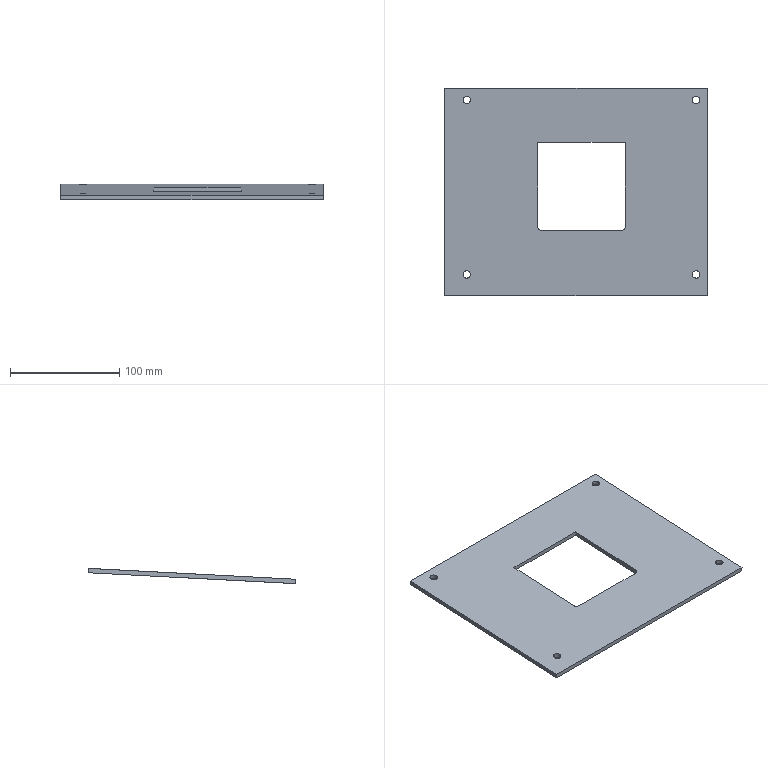Component | SolidWorks | YC1-250HangingBoxOverall-1_YC1-250SupportBracketT()-1_YC1-160OperationStationBaffleT-1 | 1 solid | 20 faces | box 240 x 189.95 x 13.94 mm | volume 155892 mm3 | cylinder 10 | plane 10 | commonest cylinder face diameters 7 x8 8 x2 | material Plain Carbon Steel
STEP:
#1=COLOUR_RGB('',0.7922,0.8196,0.9333);
#2=FILL_AREA_STYLE_COLOUR('',#1);
#3=FILL_AREA_STYLE('',(#2));
#4=SURFACE_STYLE_FILL_AREA(#3);
#5=SURFACE_SIDE_STYLE('',(#4));
#6=SURFACE_STYLE_USAGE(.BOTH.,#5);
#7=PRESENTATION_STYLE_ASSIGNMENT((#6));
#8=CARTESIAN_POINT('',(33.071,65.604,2.111));
#9=VERTEX_POINT('',#8);
#10=CARTESIAN_POINT('',(33.071,65.328,2.097));
#11=VERTEX_POINT('',#10);
#12=CARTESIAN_POINT('',(33.071,65.466,2.104));
#13=DIRECTION('',(-0.,-0.05234,0.9986));
#14=DIRECTION('',(0.,-0.9986,-0.05234));
#15=AXIS2_PLACEMENT_3D('',#12,#13,#14);
#16=CIRCLE('',#15,0.1378);
#17=EDGE_CURVE('',#9,#11,#16,.T.);
#18=ORIENTED_EDGE('',*,*,#17,.F.);
#19=CARTESIAN_POINT('',(33.071,65.595,2.268));
#20=VERTEX_POINT('',#19);
#21=CARTESIAN_POINT('',(33.071,65.604,2.111));
#22=DIRECTION('',(-0.,-0.05234,0.9986));
#23=VECTOR('',#22,39.37);
#24=LINE('',#21,#23);
#25=EDGE_CURVE('',#9,#20,#24,.T.);
#26=ORIENTED_EDGE('',*,*,#25,.T.);
#27=CARTESIAN_POINT('',(33.071,65.32,2.254));
#28=VERTEX_POINT('',#27);
#29=CARTESIAN_POINT('',(33.071,65.458,2.261));
#30=DIRECTION('',(-0.,-0.05234,0.9986));
#31=DIRECTION('',(0.,-0.9986,-0.05234));
#32=AXIS2_PLACEMENT_3D('',#29,#30,#31);
#33=CIRCLE('',#32,0.1378);
#34=EDGE_CURVE('',#20,#28,#33,.T.);
#35=ORIENTED_EDGE('',*,*,#34,.T.);
#36=CARTESIAN_POINT('',(33.071,65.328,2.097));
#37=DIRECTION('',(-0.,-0.05234,0.9986));
#38=VECTOR('',#37,39.37);
#39=LINE('',#36,#38);
#40=EDGE_CURVE('',#11,#28,#39,.T.);
#41=ORIENTED_EDGE('',*,*,#40,.F.);
#42=EDGE_LOOP('',(#18,#26,#35,#41));
#43=FACE_OUTER_BOUND('',#42,.T.);
#44=CARTESIAN_POINT('',(33.071,65.466,2.104));
#45=DIRECTION('',(-0.,-0.05234,0.9986));
#46=DIRECTION('',(0.,-0.9986,-0.05234));
#47=AXIS2_PLACEMENT_3D('',#44,#45,#46);
#48=CYLINDRICAL_SURFACE('',#47,0.1378);
#49=ADVANCED_FACE('',(#43),#48,.F.);
#50=CARTESIAN_POINT('',(41.339,65.604,2.111));
#51=VERTEX_POINT('',#50);
#52=CARTESIAN_POINT('',(41.339,65.328,2.097));
#53=VERTEX_POINT('',#52);
#54=CARTESIAN_POINT('',(41.339,65.466,2.104));
#55=DIRECTION('',(-0.,-0.05234,0.9986));
#56=DIRECTION('',(0.,-0.9986,-0.05234));
#57=AXIS2_PLACEMENT_3D('',#54,#55,#56);
#58=CIRCLE('',#57,0.1378);
#59=EDGE_CURVE('',#51,#53,#58,.T.);
#60=ORIENTED_EDGE('',*,*,#59,.F.);
#61=CARTESIAN_POINT('',(41.339,65.595,2.268));
#62=VERTEX_POINT('',#61);
#63=CARTESIAN_POINT('',(41.339,65.604,2.111));
#64=DIRECTION('',(-0.,-0.05234,0.9986));
#65=VECTOR('',#64,39.37);
#66=LINE('',#63,#65);
#67=EDGE_CURVE('',#51,#62,#66,.T.);
#68=ORIENTED_EDGE('',*,*,#67,.T.);
#69=CARTESIAN_POINT('',(41.339,65.32,2.254));
#70=VERTEX_POINT('',#69);
#71=CARTESIAN_POINT('',(41.339,65.458,2.261));
#72=DIRECTION('',(-0.,-0.05234,0.9986));
#73=DIRECTION('',(0.,-0.9986,-0.05234));
#74=AXIS2_PLACEMENT_3D('',#71,#72,#73);
#75=CIRCLE('',#74,0.1378);
#76=EDGE_CURVE('',#62,#70,#75,.T.);
#77=ORIENTED_EDGE('',*,*,#76,.T.);
#78=CARTESIAN_POINT('',(41.339,65.328,2.097));
#79=DIRECTION('',(-0.,-0.05234,0.9986));
#80=VECTOR('',#79,39.37);
#81=LINE('',#78,#80);
#82=EDGE_CURVE('',#53,#70,#81,.T.);
#83=ORIENTED_EDGE('',*,*,#82,.F.);
#84=EDGE_LOOP('',(#60,#68,#77,#83));
#85=FACE_OUTER_BOUND('',#84,.T.);
#86=CARTESIAN_POINT('',(41.339,65.466,2.104));
#87=DIRECTION('',(-0.,-0.05234,0.9986));
#88=DIRECTION('',(0.,-0.9986,-0.05234));
#89=AXIS2_PLACEMENT_3D('',#86,#87,#88);
#90=CYLINDRICAL_SURFACE('',#89,0.1378);
#91=ADVANCED_FACE('',(#85),#90,.F.);
#92=CARTESIAN_POINT('',(41.339,59.313,1.781));
#93=VERTEX_POINT('',#92);
#94=CARTESIAN_POINT('',(41.339,59.038,1.767));
#95=VERTEX_POINT('',#94);
#96=CARTESIAN_POINT('',(41.339,59.175,1.774));
#97=DIRECTION('',(-0.,-0.05234,0.9986));
#98=DIRECTION('',(0.,-0.9986,-0.05234));
#99=AXIS2_PLACEMENT_3D('',#96,#97,#98);
#100=CIRCLE('',#99,0.1378);
#101=EDGE_CURVE('',#93,#95,#100,.T.);
#102=ORIENTED_EDGE('',*,*,#101,.F.);
#103=CARTESIAN_POINT('',(41.339,59.305,1.939));
#104=VERTEX_POINT('',#103);
#105=CARTESIAN_POINT('',(41.339,59.313,1.781));
#106=DIRECTION('',(-0.,-0.05234,0.9986));
#107=VECTOR('',#106,39.37);
#108=LINE('',#105,#107);
#109=EDGE_CURVE('',#93,#104,#108,.T.);
#110=ORIENTED_EDGE('',*,*,#109,.T.);
#111=CARTESIAN_POINT('',(41.339,59.03,1.924));
#112=VERTEX_POINT('',#111);
#113=CARTESIAN_POINT('',(41.339,59.167,1.931));
#114=DIRECTION('',(-0.,-0.05234,0.9986));
#115=DIRECTION('',(0.,-0.9986,-0.05234));
#116=AXIS2_PLACEMENT_3D('',#113,#114,#115);
#117=CIRCLE('',#116,0.1378);
#118=EDGE_CURVE('',#104,#112,#117,.T.);
#119=ORIENTED_EDGE('',*,*,#118,.T.);
#120=CARTESIAN_POINT('',(41.339,59.038,1.767));
#121=DIRECTION('',(-0.,-0.05234,0.9986));
#122=VECTOR('',#121,39.37);
#123=LINE('',#120,#122);
#124=EDGE_CURVE('',#95,#112,#123,.T.);
#125=ORIENTED_EDGE('',*,*,#124,.F.);
#126=EDGE_LOOP('',(#102,#110,#119,#125));
#127=FACE_OUTER_BOUND('',#126,.T.);
#128=CARTESIAN_POINT('',(41.339,59.175,1.774));
#129=DIRECTION('',(-0.,-0.05234,0.9986));
#130=DIRECTION('',(0.,-0.9986,-0.05234));
#131=AXIS2_PLACEMENT_3D('',#128,#129,#130);
#132=CYLINDRICAL_SURFACE('',#131,0.1378);
#133=ADVANCED_FACE('',(#127),#132,.F.);
#134=CARTESIAN_POINT('',(33.071,59.313,1.781));
#135=VERTEX_POINT('',#134);
#136=CARTESIAN_POINT('',(33.071,59.038,1.767));
#137=VERTEX_POINT('',#136);
#138=CARTESIAN_POINT('',(33.071,59.175,1.774));
#139=DIRECTION('',(-0.,-0.05234,0.9986));
#140=DIRECTION('',(0.,-0.9986,-0.05234));
#141=AXIS2_PLACEMENT_3D('',#138,#139,#140);
#142=CIRCLE('',#141,0.1378);
#143=EDGE_CURVE('',#135,#137,#142,.T.);
#144=ORIENTED_EDGE('',*,*,#143,.F.);
#145=CARTESIAN_POINT('',(33.071,59.305,1.939));
#146=VERTEX_POINT('',#145);
#147=CARTESIAN_POINT('',(33.071,59.313,1.781));
#148=DIRECTION('',(-0.,-0.05234,0.9986));
#149=VECTOR('',#148,39.37);
#150=LINE('',#147,#149);
#151=EDGE_CURVE('',#135,#146,#150,.T.);
#152=ORIENTED_EDGE('',*,*,#151,.T.);
#153=CARTESIAN_POINT('',(33.071,59.03,1.924));
#154=VERTEX_POINT('',#153);
#155=CARTESIAN_POINT('',(33.071,59.167,1.931));
#156=DIRECTION('',(-0.,-0.05234,0.9986));
#157=DIRECTION('',(0.,-0.9986,-0.05234));
#158=AXIS2_PLACEMENT_3D('',#155,#156,#157);
#159=CIRCLE('',#158,0.1378);
#160=EDGE_CURVE('',#146,#154,#159,.T.);
#161=ORIENTED_EDGE('',*,*,#160,.T.);
#162=CARTESIAN_POINT('',(33.071,59.038,1.767));
#163=DIRECTION('',(-0.,-0.05234,0.9986));
#164=VECTOR('',#163,39.37);
#165=LINE('',#162,#164);
#166=EDGE_CURVE('',#137,#154,#165,.T.);
#167=ORIENTED_EDGE('',*,*,#166,.F.);
#168=EDGE_LOOP('',(#144,#152,#161,#167));
#169=FACE_OUTER_BOUND('',#168,.T.);
#170=CARTESIAN_POINT('',(33.071,59.175,1.774));
#171=DIRECTION('',(-0.,-0.05234,0.9986));
#172=DIRECTION('',(0.,-0.9986,-0.05234));
#173=AXIS2_PLACEMENT_3D('',#170,#171,#172);
#174=CYLINDRICAL_SURFACE('',#173,0.1378);
#175=ADVANCED_FACE('',(#169),#174,.F.);
#176=CARTESIAN_POINT('',(41.732,65.879,2.126));
#177=VERTEX_POINT('',#176);
#178=CARTESIAN_POINT('',(41.732,58.409,1.734));
#179=VERTEX_POINT('',#178);
#180=CARTESIAN_POINT('',(41.732,58.409,1.734));
#181=DIRECTION('',(0.,-0.9986,-0.05234));
#182=VECTOR('',#181,39.37);
#183=LINE('',#180,#182);
#184=EDGE_CURVE('',#177,#179,#183,.T.);
#185=ORIENTED_EDGE('',*,*,#184,.T.);
#186=CARTESIAN_POINT('',(32.283,58.409,1.734));
#187=VERTEX_POINT('',#186);
#188=CARTESIAN_POINT('',(32.283,58.409,1.734));
#189=DIRECTION('',(-1.,-0.,-0.));
#190=VECTOR('',#189,39.37);
#191=LINE('',#188,#190);
#192=EDGE_CURVE('',#179,#187,#191,.T.);
#193=ORIENTED_EDGE('',*,*,#192,.T.);
#194=CARTESIAN_POINT('',(32.283,65.879,2.126));
#195=VERTEX_POINT('',#194);
#196=CARTESIAN_POINT('',(32.283,58.409,1.734));
#197=DIRECTION('',(-0.,0.9986,0.05234));
#198=VECTOR('',#197,39.37);
#199=LINE('',#196,#198);
#200=EDGE_CURVE('',#187,#195,#199,.T.);
#201=ORIENTED_EDGE('',*,*,#200,.T.);
#202=CARTESIAN_POINT('',(32.283,65.879,2.126));
#203=DIRECTION('',(1.,0.,0.));
#204=VECTOR('',#203,39.37);
#205=LINE('',#202,#204);
#206=EDGE_CURVE('',#195,#177,#205,.T.);
#207=ORIENTED_EDGE('',*,*,#206,.T.);
#208=EDGE_LOOP('',(#185,#193,#201,#207));
#209=FACE_OUTER_BOUND('',#208,.T.);
#210=CARTESIAN_POINT('',(33.071,65.466,2.104));
#211=DIRECTION('',(-0.,-0.05234,0.9986));
#212=DIRECTION('',(0.,-0.9986,-0.05234));
#213=AXIS2_PLACEMENT_3D('',#210,#211,#212);
#214=CIRCLE('',#213,0.1378);
#215=EDGE_CURVE('',#11,#9,#214,.T.);
#216=ORIENTED_EDGE('',*,*,#215,.T.);
#217=ORIENTED_EDGE('',*,*,#17,.T.);
#218=EDGE_LOOP('',(#216,#217));
#219=FACE_BOUND('',#218,.T.);
#220=CARTESIAN_POINT('',(41.339,65.466,2.104));
#221=DIRECTION('',(-0.,-0.05234,0.9986));
#222=DIRECTION('',(0.,-0.9986,-0.05234));
#223=AXIS2_PLACEMENT_3D('',#220,#221,#222);
#224=CIRCLE('',#223,0.1378);
#225=EDGE_CURVE('',#53,#51,#224,.T.);
#226=ORIENTED_EDGE('',*,*,#225,.T.);
#227=ORIENTED_EDGE('',*,*,#59,.T.);
#228=EDGE_LOOP('',(#226,#227));
#229=FACE_BOUND('',#228,.T.);
#230=CARTESIAN_POINT('',(41.339,59.175,1.774));
#231=DIRECTION('',(-0.,-0.05234,0.9986));
#232=DIRECTION('',(0.,-0.9986,-0.05234));
#233=AXIS2_PLACEMENT_3D('',#230,#231,#232);
#234=CIRCLE('',#233,0.1378);
#235=EDGE_CURVE('',#95,#93,#234,.T.);
#236=ORIENTED_EDGE('',*,*,#235,.T.);
#237=ORIENTED_EDGE('',*,*,#101,.T.);
#238=EDGE_LOOP('',(#236,#237));
#239=FACE_BOUND('',#238,.T.);
#240=CARTESIAN_POINT('',(33.071,59.175,1.774));
#241=DIRECTION('',(-0.,-0.05234,0.9986));
#242=DIRECTION('',(0.,-0.9986,-0.05234));
#243=AXIS2_PLACEMENT_3D('',#240,#241,#242);
#244=CIRCLE('',#243,0.1378);
#245=EDGE_CURVE('',#137,#135,#244,.T.);
#246=ORIENTED_EDGE('',*,*,#245,.T.);
#247=ORIENTED_EDGE('',*,*,#143,.T.);
#248=EDGE_LOOP('',(#246,#247));
#249=FACE_BOUND('',#248,.T.);
#250=CARTESIAN_POINT('',(38.78,63.933,2.024));
#251=VERTEX_POINT('',#250);
#252=CARTESIAN_POINT('',(35.63,63.933,2.024));
#253=VERTEX_POINT('',#252);
#254=CARTESIAN_POINT('',(32.283,63.933,2.024));
#255=DIRECTION('',(-1.,-0.,-0.));
#256=VECTOR('',#255,39.37);
#257=LINE('',#254,#256);
#258=EDGE_CURVE('',#251,#253,#257,.T.);
#259=ORIENTED_EDGE('',*,*,#258,.T.);
#260=CARTESIAN_POINT('',(35.63,60.905,1.865));
#261=VERTEX_POINT('',#260);
#262=CARTESIAN_POINT('',(35.63,63.893,2.021));
#263=DIRECTION('',(-0.,0.9986,0.05234));
#264=VECTOR('',#263,39.37);
#265=LINE('',#262,#264);
#266=EDGE_CURVE('',#261,#253,#265,.T.);
#267=ORIENTED_EDGE('',*,*,#266,.F.);
#268=CARTESIAN_POINT('',(35.787,60.748,1.857));
#269=VERTEX_POINT('',#268);
#270=CARTESIAN_POINT('',(35.787,60.905,1.865));
#271=DIRECTION('',(-0.,-0.05234,0.9986));
#272=DIRECTION('',(0.,-0.9986,-0.05234));
#273=AXIS2_PLACEMENT_3D('',#270,#271,#272);
#274=CIRCLE('',#273,0.1575);
#275=EDGE_CURVE('',#261,#269,#274,.T.);
#276=ORIENTED_EDGE('',*,*,#275,.T.);
#277=CARTESIAN_POINT('',(38.622,60.748,1.857));
#278=VERTEX_POINT('',#277);
#279=CARTESIAN_POINT('',(35.63,60.748,1.857));
#280=DIRECTION('',(-1.,-0.,-0.));
#281=VECTOR('',#280,39.37);
#282=LINE('',#279,#281);
#283=EDGE_CURVE('',#278,#269,#282,.T.);
#284=ORIENTED_EDGE('',*,*,#283,.F.);
#285=CARTESIAN_POINT('',(38.78,60.905,1.865));
#286=VERTEX_POINT('',#285);
#287=CARTESIAN_POINT('',(38.622,60.905,1.865));
#288=DIRECTION('',(-0.,-0.05234,0.9986));
#289=DIRECTION('',(0.,-0.9986,-0.05234));
#290=AXIS2_PLACEMENT_3D('',#287,#288,#289);
#291=CIRCLE('',#290,0.1575);
#292=EDGE_CURVE('',#278,#286,#291,.T.);
#293=ORIENTED_EDGE('',*,*,#292,.T.);
#294=CARTESIAN_POINT('',(38.78,63.893,2.021));
#295=DIRECTION('',(0.,-0.9986,-0.05234));
#296=VECTOR('',#295,39.37);
#297=LINE('',#294,#296);
#298=EDGE_CURVE('',#251,#286,#297,.T.);
#299=ORIENTED_EDGE('',*,*,#298,.F.);
#300=EDGE_LOOP('',(#259,#267,#276,#284,#293,#299));
#301=FACE_BOUND('',#300,.T.);
#302=CARTESIAN_POINT('',(32.283,65.879,2.126));
#303=DIRECTION('',(0.,0.05234,-0.9986));
#304=DIRECTION('',(-0.,0.9986,0.05234));
#305=AXIS2_PLACEMENT_3D('',#302,#303,#304);
#306=PLANE('',#305);
#307=ADVANCED_FACE('',(#209,#219,#229,#239,#249,#301),#306,.T.);
#308=CARTESIAN_POINT('',(33.071,59.167,1.931));
#309=DIRECTION('',(-0.,-0.05234,0.9986));
#310=DIRECTION('',(0.,-0.9986,-0.05234));
#311=AXIS2_PLACEMENT_3D('',#308,#309,#310);
#312=CIRCLE('',#311,0.1378);
#313=EDGE_CURVE('',#154,#146,#312,.T.);
#314=ORIENTED_EDGE('',*,*,#313,.F.);
#315=ORIENTED_EDGE('',*,*,#160,.F.);
#316=EDGE_LOOP('',(#314,#315));
#317=FACE_BOUND('',#316,.T.);
#318=CARTESIAN_POINT('',(41.339,59.167,1.931));
#319=DIRECTION('',(-0.,-0.05234,0.9986));
#320=DIRECTION('',(0.,-0.9986,-0.05234));
#321=AXIS2_PLACEMENT_3D('',#318,#319,#320);
#322=CIRCLE('',#321,0.1378);
#323=EDGE_CURVE('',#112,#104,#322,.T.);
#324=ORIENTED_EDGE('',*,*,#323,.F.);
#325=ORIENTED_EDGE('',*,*,#118,.F.);
#326=EDGE_LOOP('',(#324,#325));
#327=FACE_BOUND('',#326,.T.);
#328=CARTESIAN_POINT('',(41.339,65.458,2.261));
#329=DIRECTION('',(-0.,-0.05234,0.9986));
#330=DIRECTION('',(0.,-0.9986,-0.05234));
#331=AXIS2_PLACEMENT_3D('',#328,#329,#330);
#332=CIRCLE('',#331,0.1378);
#333=EDGE_CURVE('',#70,#62,#332,.T.);
#334=ORIENTED_EDGE('',*,*,#333,.F.);
#335=ORIENTED_EDGE('',*,*,#76,.F.);
#336=EDGE_LOOP('',(#334,#335));
#337=FACE_BOUND('',#336,.T.);
#338=CARTESIAN_POINT('',(33.071,65.458,2.261));
#339=DIRECTION('',(-0.,-0.05234,0.9986));
#340=DIRECTION('',(0.,-0.9986,-0.05234));
#341=AXIS2_PLACEMENT_3D('',#338,#339,#340);
#342=CIRCLE('',#341,0.1378);
#343=EDGE_CURVE('',#28,#20,#342,.T.);
#344=ORIENTED_EDGE('',*,*,#343,.F.);
#345=ORIENTED_EDGE('',*,*,#34,.F.);
#346=EDGE_LOOP('',(#344,#345));
#347=FACE_BOUND('',#346,.T.);
#348=CARTESIAN_POINT('',(41.732,58.4,1.891));
#349=VERTEX_POINT('',#348);
#350=CARTESIAN_POINT('',(32.283,58.4,1.891));
#351=VERTEX_POINT('',#350);
#352=CARTESIAN_POINT('',(32.283,58.4,1.891));
#353=DIRECTION('',(-1.,-0.,-0.));
#354=VECTOR('',#353,39.37);
#355=LINE('',#352,#354);
#356=EDGE_CURVE('',#349,#351,#355,.T.);
#357=ORIENTED_EDGE('',*,*,#356,.F.);
#358=CARTESIAN_POINT('',(41.732,65.871,2.283));
#359=VERTEX_POINT('',#358);
#360=CARTESIAN_POINT('',(41.732,65.871,2.283));
#361=DIRECTION('',(0.,-0.9986,-0.05234));
#362=VECTOR('',#361,39.37);
#363=LINE('',#360,#362);
#364=EDGE_CURVE('',#359,#349,#363,.T.);
#365=ORIENTED_EDGE('',*,*,#364,.F.);
#366=CARTESIAN_POINT('',(32.283,65.871,2.283));
#367=VERTEX_POINT('',#366);
#368=CARTESIAN_POINT('',(32.283,65.871,2.283));
#369=DIRECTION('',(1.,0.,0.));
#370=VECTOR('',#369,39.37);
#371=LINE('',#368,#370);
#372=EDGE_CURVE('',#367,#359,#371,.T.);
#373=ORIENTED_EDGE('',*,*,#372,.F.);
#374=CARTESIAN_POINT('',(32.283,65.871,2.283));
#375=DIRECTION('',(-0.,0.9986,0.05234));
#376=VECTOR('',#375,39.37);
#377=LINE('',#374,#376);
#378=EDGE_CURVE('',#351,#367,#377,.T.);
#379=ORIENTED_EDGE('',*,*,#378,.F.);
#380=EDGE_LOOP('',(#357,#365,#373,#379));
#381=FACE_OUTER_BOUND('',#380,.T.);
#382=CARTESIAN_POINT('',(35.63,63.924,2.181));
#383=VERTEX_POINT('',#382);
#384=CARTESIAN_POINT('',(35.63,60.897,2.022));
#385=VERTEX_POINT('',#384);
#386=CARTESIAN_POINT('',(35.63,65.871,2.283));
#387=DIRECTION('',(0.,-0.9986,-0.05234));
#388=VECTOR('',#387,39.37);
#389=LINE('',#386,#388);
#390=EDGE_CURVE('',#383,#385,#389,.T.);
#391=ORIENTED_EDGE('',*,*,#390,.F.);
#392=CARTESIAN_POINT('',(38.78,63.924,2.181));
#393=VERTEX_POINT('',#392);
#394=CARTESIAN_POINT('',(38.78,63.924,2.181));
#395=DIRECTION('',(-1.,-0.,-0.));
#396=VECTOR('',#395,39.37);
#397=LINE('',#394,#396);
#398=EDGE_CURVE('',#393,#383,#397,.T.);
#399=ORIENTED_EDGE('',*,*,#398,.F.);
#400=CARTESIAN_POINT('',(38.78,60.897,2.022));
#401=VERTEX_POINT('',#400);
#402=CARTESIAN_POINT('',(38.78,65.871,2.283));
#403=DIRECTION('',(-0.,0.9986,0.05234));
#404=VECTOR('',#403,39.37);
#405=LINE('',#402,#404);
#406=EDGE_CURVE('',#401,#393,#405,.T.);
#407=ORIENTED_EDGE('',*,*,#406,.F.);
#408=CARTESIAN_POINT('',(38.622,60.74,2.014));
#409=VERTEX_POINT('',#408);
#410=CARTESIAN_POINT('',(38.622,60.897,2.022));
#411=DIRECTION('',(-0.,-0.05234,0.9986));
#412=DIRECTION('',(0.,-0.9986,-0.05234));
#413=AXIS2_PLACEMENT_3D('',#410,#411,#412);
#414=CIRCLE('',#413,0.1575);
#415=EDGE_CURVE('',#409,#401,#414,.T.);
#416=ORIENTED_EDGE('',*,*,#415,.F.);
#417=CARTESIAN_POINT('',(35.787,60.74,2.014));
#418=VERTEX_POINT('',#417);
#419=CARTESIAN_POINT('',(32.283,60.74,2.014));
#420=DIRECTION('',(1.,0.,0.));
#421=VECTOR('',#420,39.37);
#422=LINE('',#419,#421);
#423=EDGE_CURVE('',#418,#409,#422,.T.);
#424=ORIENTED_EDGE('',*,*,#423,.F.);
#425=CARTESIAN_POINT('',(35.787,60.897,2.022));
#426=DIRECTION('',(-0.,-0.05234,0.9986));
#427=DIRECTION('',(0.,-0.9986,-0.05234));
#428=AXIS2_PLACEMENT_3D('',#425,#426,#427);
#429=CIRCLE('',#428,0.1575);
#430=EDGE_CURVE('',#385,#418,#429,.T.);
#431=ORIENTED_EDGE('',*,*,#430,.F.);
#432=EDGE_LOOP('',(#391,#399,#407,#416,#424,#431));
#433=FACE_BOUND('',#432,.T.);
#434=CARTESIAN_POINT('',(32.283,65.871,2.283));
#435=DIRECTION('',(0.,0.05234,-0.9986));
#436=DIRECTION('',(-0.,0.9986,0.05234));
#437=AXIS2_PLACEMENT_3D('',#434,#435,#436);
#438=PLANE('',#437);
#439=ADVANCED_FACE('',(#317,#327,#337,#347,#381,#433),#438,.F.);
#440=ORIENTED_EDGE('',*,*,#390,.T.);
#441=CARTESIAN_POINT('',(35.63,60.897,2.022));
#442=DIRECTION('',(0.,0.05234,-0.9986));
#443=VECTOR('',#442,39.37);
#444=LINE('',#441,#443);
#445=EDGE_CURVE('',#385,#261,#444,.T.);
#446=ORIENTED_EDGE('',*,*,#445,.T.);
#447=ORIENTED_EDGE('',*,*,#266,.T.);
#448=CARTESIAN_POINT('',(35.63,63.933,2.024));
#449=DIRECTION('',(-0.,-0.05234,0.9986));
#450=VECTOR('',#449,39.37);
#451=LINE('',#448,#450);
#452=EDGE_CURVE('',#253,#383,#451,.T.);
#453=ORIENTED_EDGE('',*,*,#452,.T.);
#454=EDGE_LOOP('',(#440,#446,#447,#453));
#455=FACE_OUTER_BOUND('',#454,.T.);
#456=CARTESIAN_POINT('',(35.63,63.885,2.179));
#457=DIRECTION('',(1.,0.,0.));
#458=DIRECTION('',(-0.,0.9986,0.05234));
#459=AXIS2_PLACEMENT_3D('',#456,#457,#458);
#460=PLANE('',#459);
#461=ADVANCED_FACE('',(#455),#460,.T.);
#462=ORIENTED_EDGE('',*,*,#406,.T.);
#463=CARTESIAN_POINT('',(38.78,63.933,2.024));
#464=DIRECTION('',(-0.,-0.05234,0.9986));
#465=VECTOR('',#464,39.37);
#466=LINE('',#463,#465);
#467=EDGE_CURVE('',#251,#393,#466,.T.);
#468=ORIENTED_EDGE('',*,*,#467,.F.);
#469=ORIENTED_EDGE('',*,*,#298,.T.);
#470=CARTESIAN_POINT('',(38.78,60.897,2.022));
#471=DIRECTION('',(-0.,-0.05234,0.9986));
#472=VECTOR('',#471,39.37);
#473=LINE('',#470,#472);
#474=EDGE_CURVE('',#286,#401,#473,.T.);
#475=ORIENTED_EDGE('',*,*,#474,.T.);
#476=EDGE_LOOP('',(#462,#468,#469,#475));
#477=FACE_OUTER_BOUND('',#476,.T.);
#478=CARTESIAN_POINT('',(38.78,63.885,2.179));
#479=DIRECTION('',(-1.,-0.,-0.));
#480=DIRECTION('',(-0.,-0.05234,0.9986));
#481=AXIS2_PLACEMENT_3D('',#478,#479,#480);
#482=PLANE('',#481);
#483=ADVANCED_FACE('',(#477),#482,.T.);
#484=ORIENTED_EDGE('',*,*,#474,.F.);
#485=ORIENTED_EDGE('',*,*,#292,.F.);
#486=CARTESIAN_POINT('',(38.622,60.74,2.014));
#487=DIRECTION('',(0.,0.05234,-0.9986));
#488=VECTOR('',#487,39.37);
#489=LINE('',#486,#488);
#490=EDGE_CURVE('',#409,#278,#489,.T.);
#491=ORIENTED_EDGE('',*,*,#490,.F.);
#492=ORIENTED_EDGE('',*,*,#415,.T.);
#493=EDGE_LOOP('',(#484,#485,#491,#492));
#494=FACE_OUTER_BOUND('',#493,.T.);
#495=CARTESIAN_POINT('',(38.622,60.897,2.022));
#496=DIRECTION('',(-0.,-0.05234,0.9986));
#497=DIRECTION('',(0.,-0.9986,-0.05234));
#498=AXIS2_PLACEMENT_3D('',#495,#496,#497);
#499=CYLINDRICAL_SURFACE('',#498,0.1575);
#500=ADVANCED_FACE('',(#494),#499,.F.);
#501=ORIENTED_EDGE('',*,*,#283,.T.);
#502=CARTESIAN_POINT('',(35.787,60.74,2.014));
#503=DIRECTION('',(-0.,-0.05234,0.9986));
#504=VECTOR('',#503,39.37);
#505=LINE('',#502,#504);
#506=EDGE_CURVE('',#269,#418,#505,.T.);
#507=ORIENTED_EDGE('',*,*,#506,.T.);
#508=ORIENTED_EDGE('',*,*,#423,.T.);
#509=ORIENTED_EDGE('',*,*,#490,.T.);
#510=EDGE_LOOP('',(#501,#507,#508,#509));
#511=FACE_OUTER_BOUND('',#510,.T.);
#512=CARTESIAN_POINT('',(35.63,60.74,2.014));
#513=DIRECTION('',(-0.,0.9986,0.05234));
#514=DIRECTION('',(-0.,-0.05234,0.9986));
#515=AXIS2_PLACEMENT_3D('',#512,#513,#514);
#516=PLANE('',#515);
#517=ADVANCED_FACE('',(#511),#516,.T.);
#518=ORIENTED_EDGE('',*,*,#506,.F.);
#519=ORIENTED_EDGE('',*,*,#275,.F.);
#520=ORIENTED_EDGE('',*,*,#445,.F.);
#521=ORIENTED_EDGE('',*,*,#430,.T.);
#522=EDGE_LOOP('',(#518,#519,#520,#521));
#523=FACE_OUTER_BOUND('',#522,.T.);
#524=CARTESIAN_POINT('',(35.787,60.897,2.022));
#525=DIRECTION('',(-0.,-0.05234,0.9986));
#526=DIRECTION('',(0.,-0.9986,-0.05234));
#527=AXIS2_PLACEMENT_3D('',#524,#525,#526);
#528=CYLINDRICAL_SURFACE('',#527,0.1575);
#529=ADVANCED_FACE('',(#523),#528,.F.);
#530=CARTESIAN_POINT('',(32.283,58.4,1.891));
#531=DIRECTION('',(0.,0.05234,-0.9986));
#532=VECTOR('',#531,39.37);
#533=LINE('',#530,#532);
#534=EDGE_CURVE('',#351,#187,#533,.T.);
#535=ORIENTED_EDGE('',*,*,#534,.F.);
#536=ORIENTED_EDGE('',*,*,#378,.T.);
#537=CARTESIAN_POINT('',(32.283,65.871,2.283));
#538=DIRECTION('',(-0.,-0.05234,0.9986));
#539=VECTOR('',#538,39.37);
#540=LINE('',#537,#539);
#541=EDGE_CURVE('',#195,#367,#540,.T.);
#542=ORIENTED_EDGE('',*,*,#541,.F.);
#543=ORIENTED_EDGE('',*,*,#200,.F.);
#544=EDGE_LOOP('',(#535,#536,#542,#543));
#545=FACE_OUTER_BOUND('',#544,.T.);
#546=CARTESIAN_POINT('',(32.283,58.4,1.891));
#547=DIRECTION('',(1.,0.,0.));
#548=DIRECTION('',(0.,0.05234,-0.9986));
#549=AXIS2_PLACEMENT_3D('',#546,#547,#548);
#550=PLANE('',#549);
#551=ADVANCED_FACE('',(#545),#550,.F.);
#552=CARTESIAN_POINT('',(41.732,58.4,1.891));
#553=DIRECTION('',(0.,0.05234,-0.9986));
#554=VECTOR('',#553,39.37);
#555=LINE('',#552,#554);
#556=EDGE_CURVE('',#349,#179,#555,.T.);
#557=ORIENTED_EDGE('',*,*,#556,.F.);
#558=ORIENTED_EDGE('',*,*,#356,.T.);
#559=ORIENTED_EDGE('',*,*,#534,.T.);
#560=ORIENTED_EDGE('',*,*,#192,.F.);
#561=EDGE_LOOP('',(#557,#558,#559,#560));
#562=FACE_OUTER_BOUND('',#561,.T.);
#563=CARTESIAN_POINT('',(32.283,58.4,1.891));
#564=DIRECTION('',(-0.,0.9986,0.05234));
#565=DIRECTION('',(-0.,-0.05234,0.9986));
#566=AXIS2_PLACEMENT_3D('',#563,#564,#565);
#567=PLANE('',#566);
#568=ADVANCED_FACE('',(#562),#567,.F.);
#569=CARTESIAN_POINT('',(41.732,65.871,2.283));
#570=DIRECTION('',(0.,0.05234,-0.9986));
#571=VECTOR('',#570,39.37);
#572=LINE('',#569,#571);
#573=EDGE_CURVE('',#359,#177,#572,.T.);
#574=ORIENTED_EDGE('',*,*,#573,.F.);
#575=ORIENTED_EDGE('',*,*,#364,.T.);
#576=ORIENTED_EDGE('',*,*,#556,.T.);
#577=ORIENTED_EDGE('',*,*,#184,.F.);
#578=EDGE_LOOP('',(#574,#575,#576,#577));
#579=FACE_OUTER_BOUND('',#578,.T.);
#580=CARTESIAN_POINT('',(41.732,58.4,1.891));
#581=DIRECTION('',(-1.,-0.,-0.));
#582=DIRECTION('',(-0.,-0.05234,0.9986));
#583=AXIS2_PLACEMENT_3D('',#580,#581,#582);
#584=PLANE('',#583);
#585=ADVANCED_FACE('',(#579),#584,.F.);
#586=ORIENTED_EDGE('',*,*,#541,.T.);
#587=ORIENTED_EDGE('',*,*,#372,.T.);
#588=ORIENTED_EDGE('',*,*,#573,.T.);
#589=ORIENTED_EDGE('',*,*,#206,.F.);
#590=EDGE_LOOP('',(#586,#587,#588,#589));
#591=FACE_OUTER_BOUND('',#590,.T.);
#592=CARTESIAN_POINT('',(32.283,65.871,2.283));
#593=DIRECTION('',(0.,-0.9986,-0.05234));
#594=DIRECTION('',(0.,0.05234,-0.9986));
#595=AXIS2_PLACEMENT_3D('',#592,#593,#594);
#596=PLANE('',#595);
#597=ADVANCED_FACE('',(#591),#596,.F.);
#598=ORIENTED_EDGE('',*,*,#25,.F.);
#599=ORIENTED_EDGE('',*,*,#215,.F.);
#600=ORIENTED_EDGE('',*,*,#40,.T.);
#601=ORIENTED_EDGE('',*,*,#343,.T.);
#602=EDGE_LOOP('',(#598,#599,#600,#601));
#603=FACE_OUTER_BOUND('',#602,.T.);
#604=CARTESIAN_POINT('',(33.071,65.466,2.104));
#605=DIRECTION('',(-0.,-0.05234,0.9986));
#606=DIRECTION('',(0.,-0.9986,-0.05234));
#607=AXIS2_PLACEMENT_3D('',#604,#605,#606);
#608=CYLINDRICAL_SURFACE('',#607,0.1378);
#609=ADVANCED_FACE('',(#603),#608,.F.);
#610=ORIENTED_EDGE('',*,*,#67,.F.);
#611=ORIENTED_EDGE('',*,*,#225,.F.);
#612=ORIENTED_EDGE('',*,*,#82,.T.);
#613=ORIENTED_EDGE('',*,*,#333,.T.);
#614=EDGE_LOOP('',(#610,#611,#612,#613));
#615=FACE_OUTER_BOUND('',#614,.T.);
#616=CARTESIAN_POINT('',(41.339,65.466,2.104));
#617=DIRECTION('',(-0.,-0.05234,0.9986));
#618=DIRECTION('',(0.,-0.9986,-0.05234));
#619=AXIS2_PLACEMENT_3D('',#616,#617,#618);
#620=CYLINDRICAL_SURFACE('',#619,0.1378);
#621=ADVANCED_FACE('',(#615),#620,.F.);
#622=ORIENTED_EDGE('',*,*,#109,.F.);
#623=ORIENTED_EDGE('',*,*,#235,.F.);
#624=ORIENTED_EDGE('',*,*,#124,.T.);
#625=ORIENTED_EDGE('',*,*,#323,.T.);
#626=EDGE_LOOP('',(#622,#623,#624,#625));
#627=FACE_OUTER_BOUND('',#626,.T.);
#628=CARTESIAN_POINT('',(41.339,59.175,1.774));
#629=DIRECTION('',(-0.,-0.05234,0.9986));
#630=DIRECTION('',(0.,-0.9986,-0.05234));
#631=AXIS2_PLACEMENT_3D('',#628,#629,#630);
#632=CYLINDRICAL_SURFACE('',#631,0.1378);
#633=ADVANCED_FACE('',(#627),#632,.F.);
#634=ORIENTED_EDGE('',*,*,#151,.F.);
#635=ORIENTED_EDGE('',*,*,#245,.F.);
#636=ORIENTED_EDGE('',*,*,#166,.T.);
#637=ORIENTED_EDGE('',*,*,#313,.T.);
#638=EDGE_LOOP('',(#634,#635,#636,#637));
#639=FACE_OUTER_BOUND('',#638,.T.);
#640=CARTESIAN_POINT('',(33.071,59.175,1.774));
#641=DIRECTION('',(-0.,-0.05234,0.9986));
#642=DIRECTION('',(0.,-0.9986,-0.05234));
#643=AXIS2_PLACEMENT_3D('',#640,#641,#642);
#644=CYLINDRICAL_SURFACE('',#643,0.1378);
#645=ADVANCED_FACE('',(#639),#644,.F.);
#646=ORIENTED_EDGE('',*,*,#452,.F.);
#647=ORIENTED_EDGE('',*,*,#258,.F.);
#648=ORIENTED_EDGE('',*,*,#467,.T.);
#649=ORIENTED_EDGE('',*,*,#398,.T.);
#650=EDGE_LOOP('',(#646,#647,#648,#649));
#651=FACE_OUTER_BOUND('',#650,.T.);
#652=CARTESIAN_POINT('',(38.78,63.933,2.024));
#653=DIRECTION('',(-0.,0.9986,0.05234));
#654=DIRECTION('',(-0.,-0.05234,0.9986));
#655=AXIS2_PLACEMENT_3D('',#652,#653,#654);
#656=PLANE('',#655);
#657=ADVANCED_FACE('',(#651),#656,.F.);
#658=CLOSED_SHELL('',(#49,#91,#133,#175,#307,#439,#461,#483,#500,#517,#529,#551,#568,#585,#597,#609,#621,#633,#645,#657));
#659=MANIFOLD_SOLID_BREP('',#658);
#660=STYLED_ITEM('',(#7),#659);
#661=(LENGTH_UNIT()NAMED_UNIT(*)SI_UNIT($,.METRE.));
#662=LENGTH_MEASURE_WITH_UNIT(LENGTH_MEASURE(0.0254),#661);
#663=DIMENSIONAL_EXPONENTS(1.,0.,0.,0.,0.,0.,0.);
#664=(CONVERSION_BASED_UNIT('',#662)LENGTH_UNIT()NAMED_UNIT(#663));
#665=UNCERTAINTY_MEASURE_WITH_UNIT(LENGTH_MEASURE(0.00001),#664,'','');
#666=(NAMED_UNIT(*)PLANE_ANGLE_UNIT()SI_UNIT($,.RADIAN.));
#667=(NAMED_UNIT(*)SI_UNIT($,.STERADIAN.)SOLID_ANGLE_UNIT());
#668=(GEOMETRIC_REPRESENTATION_CONTEXT(3)GLOBAL_UNCERTAINTY_ASSIGNED_CONTEXT((#665))GLOBAL_UNIT_ASSIGNED_CONTEXT((#664,#666,#667))REPRESENTATION_CONTEXT('',''));
#669=MECHANICAL_DESIGN_GEOMETRIC_PRESENTATION_REPRESENTATION('',(#660),#668);
#670=PRESENTATION_LAYER_ASSIGNMENT('','',(#660));
#671=CARTESIAN_POINT('',(0.,0.,0.));
#672=DIRECTION('',(0.,0.,1.));
#673=DIRECTION('',(1.,0.,0.));
#674=AXIS2_PLACEMENT_3D('',#671,#672,#673);
#675=(LENGTH_UNIT()NAMED_UNIT(*)SI_UNIT($,.METRE.));
#676=LENGTH_MEASURE_WITH_UNIT(LENGTH_MEASURE(0.0254),#675);
#677=DIMENSIONAL_EXPONENTS(1.,0.,0.,0.,0.,0.,0.);
#678=(CONVERSION_BASED_UNIT('',#676)LENGTH_UNIT()NAMED_UNIT(#677));
#679=UNCERTAINTY_MEASURE_WITH_UNIT(LENGTH_MEASURE(0.00001),#678,'','');
#680=(NAMED_UNIT(*)PLANE_ANGLE_UNIT()SI_UNIT($,.RADIAN.));
#681=(NAMED_UNIT(*)SI_UNIT($,.STERADIAN.)SOLID_ANGLE_UNIT());
#682=(GEOMETRIC_REPRESENTATION_CONTEXT(3)GLOBAL_UNCERTAINTY_ASSIGNED_CONTEXT((#679))GLOBAL_UNIT_ASSIGNED_CONTEXT((#678,#680,#681))REPRESENTATION_CONTEXT('',''));
#683=ADVANCED_BREP_SHAPE_REPRESENTATION('',(#659,#674),#682);